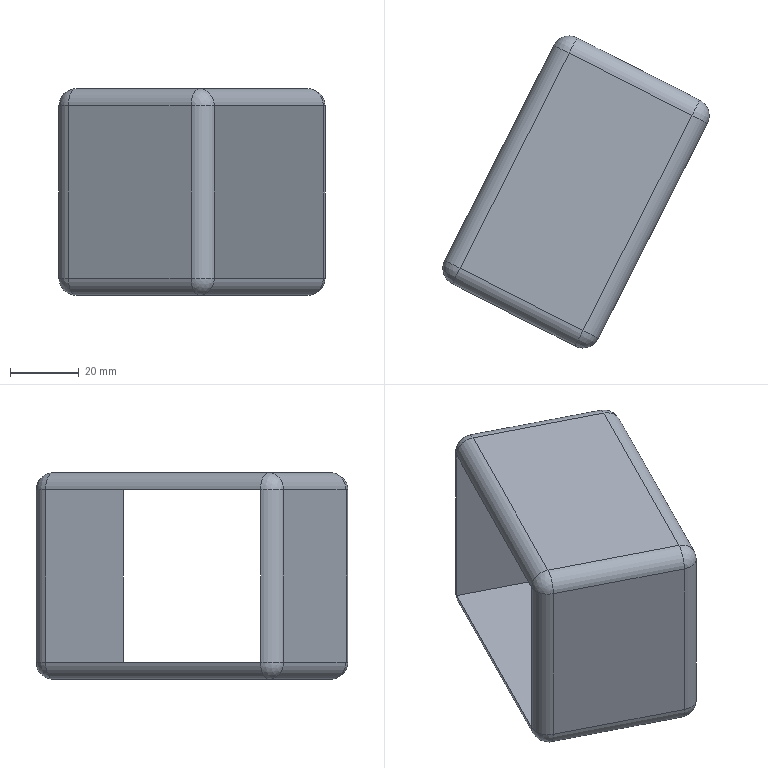Component | SolidWorks | FrameAssemblyDrawing11111-1_Part5ConnectingSleeve-1 | 1 solid | 28 faces | box 77.33 x 90.52 x 60 mm | volume 61090 mm3 | cylinder 12 | sphere 8 | plane 8 | commonest cylinder face diameters 10 x12
STEP:
#1=COLOUR_RGB('',0.7922,0.8196,0.9333);
#2=FILL_AREA_STYLE_COLOUR('',#1);
#3=FILL_AREA_STYLE('',(#2));
#4=SURFACE_STYLE_FILL_AREA(#3);
#5=SURFACE_SIDE_STYLE('',(#4));
#6=SURFACE_STYLE_USAGE(.BOTH.,#5);
#7=PRESENTATION_STYLE_ASSIGNMENT((#6));
#8=CARTESIAN_POINT('',(-32.016,-14.083,42.755));
#9=VERTEX_POINT('',#8);
#10=CARTESIAN_POINT('',(-32.28,-14.169,42.755));
#11=VERTEX_POINT('',#10);
#12=CARTESIAN_POINT('',(-32.105,-14.258,42.755));
#13=DIRECTION('',(-0.,-0.,1.));
#14=DIRECTION('',(0.892,-0.4521,-0.));
#15=AXIS2_PLACEMENT_3D('',#12,#13,#14);
#16=CIRCLE('',#15,0.1969);
#17=EDGE_CURVE('',#9,#11,#16,.T.);
#18=ORIENTED_EDGE('',*,*,#17,.F.);
#19=CARTESIAN_POINT('',(-32.016,-14.083,40.786));
#20=VERTEX_POINT('',#19);
#21=CARTESIAN_POINT('',(-32.016,-14.083,42.952));
#22=DIRECTION('',(-0.,-0.,1.));
#23=VECTOR('',#22,39.37);
#24=LINE('',#21,#23);
#25=EDGE_CURVE('',#20,#9,#24,.T.);
#26=ORIENTED_EDGE('',*,*,#25,.F.);
#27=CARTESIAN_POINT('',(-32.28,-14.169,40.786));
#28=VERTEX_POINT('',#27);
#29=CARTESIAN_POINT('',(-32.105,-14.258,40.786));
#30=DIRECTION('',(-0.,-0.,1.));
#31=DIRECTION('',(0.892,-0.4521,-0.));
#32=AXIS2_PLACEMENT_3D('',#29,#30,#31);
#33=CIRCLE('',#32,0.1969);
#34=EDGE_CURVE('',#20,#28,#33,.T.);
#35=ORIENTED_EDGE('',*,*,#34,.T.);
#36=CARTESIAN_POINT('',(-32.28,-14.169,42.952));
#37=DIRECTION('',(0.,0.,-1.));
#38=VECTOR('',#37,39.37);
#39=LINE('',#36,#38);
#40=EDGE_CURVE('',#11,#28,#39,.T.);
#41=ORIENTED_EDGE('',*,*,#40,.F.);
#42=EDGE_LOOP('',(#18,#26,#35,#41));
#43=FACE_OUTER_BOUND('',#42,.T.);
#44=CARTESIAN_POINT('',(-32.105,-14.258,42.952));
#45=DIRECTION('',(0.,0.,-1.));
#46=DIRECTION('',(-0.892,0.4521,0.));
#47=AXIS2_PLACEMENT_3D('',#44,#45,#46);
#48=CYLINDRICAL_SURFACE('',#47,0.1969);
#49=ADVANCED_FACE('',(#43),#48,.T.);
#50=ORIENTED_EDGE('',*,*,#34,.F.);
#51=CARTESIAN_POINT('',(-32.105,-14.258,40.589));
#52=VERTEX_POINT('',#51);
#53=CARTESIAN_POINT('',(-32.105,-14.258,40.786));
#54=DIRECTION('',(0.892,-0.4521,-0.));
#55=DIRECTION('',(-0.,-0.,1.));
#56=AXIS2_PLACEMENT_3D('',#53,#54,#55);
#57=CIRCLE('',#56,0.1969);
#58=EDGE_CURVE('',#52,#20,#57,.T.);
#59=ORIENTED_EDGE('',*,*,#58,.F.);
#60=CARTESIAN_POINT('',(-32.105,-14.258,40.786));
#61=DIRECTION('',(0.4521,0.892,0.));
#62=DIRECTION('',(-0.,-0.,1.));
#63=AXIS2_PLACEMENT_3D('',#60,#61,#62);
#64=CIRCLE('',#63,0.1969);
#65=EDGE_CURVE('',#52,#28,#64,.T.);
#66=ORIENTED_EDGE('',*,*,#65,.T.);
#67=EDGE_LOOP('',(#50,#59,#66));
#68=FACE_OUTER_BOUND('',#67,.T.);
#69=CARTESIAN_POINT('',(-32.105,-14.258,40.786));
#70=DIRECTION('',(0.4521,0.892,0.));
#71=DIRECTION('',(-0.,-0.,1.));
#72=AXIS2_PLACEMENT_3D('',#69,#70,#71);
#73=SPHERICAL_SURFACE('',#72,0.1969);
#74=ADVANCED_FACE('',(#68),#73,.T.);
#75=ORIENTED_EDGE('',*,*,#65,.F.);
#76=CARTESIAN_POINT('',(-33.351,-16.717,40.589));
#77=VERTEX_POINT('',#76);
#78=CARTESIAN_POINT('',(-32.016,-14.083,40.589));
#79=DIRECTION('',(0.4521,0.892,0.));
#80=VECTOR('',#79,39.37);
#81=LINE('',#78,#80);
#82=EDGE_CURVE('',#77,#52,#81,.T.);
#83=ORIENTED_EDGE('',*,*,#82,.F.);
#84=CARTESIAN_POINT('',(-33.526,-16.628,40.786));
#85=VERTEX_POINT('',#84);
#86=CARTESIAN_POINT('',(-33.351,-16.717,40.786));
#87=DIRECTION('',(0.4521,0.892,0.));
#88=DIRECTION('',(-0.,-0.,1.));
#89=AXIS2_PLACEMENT_3D('',#86,#87,#88);
#90=CIRCLE('',#89,0.1969);
#91=EDGE_CURVE('',#77,#85,#90,.T.);
#92=ORIENTED_EDGE('',*,*,#91,.T.);
#93=CARTESIAN_POINT('',(-32.191,-13.994,40.786));
#94=DIRECTION('',(-0.4521,-0.892,-0.));
#95=VECTOR('',#94,39.37);
#96=LINE('',#93,#95);
#97=EDGE_CURVE('',#28,#85,#96,.T.);
#98=ORIENTED_EDGE('',*,*,#97,.F.);
#99=EDGE_LOOP('',(#75,#83,#92,#98));
#100=FACE_OUTER_BOUND('',#99,.T.);
#101=CARTESIAN_POINT('',(-32.016,-14.083,40.786));
#102=DIRECTION('',(-0.4521,-0.892,-0.));
#103=DIRECTION('',(0.,0.,-1.));
#104=AXIS2_PLACEMENT_3D('',#101,#102,#103);
#105=CYLINDRICAL_SURFACE('',#104,0.1969);
#106=ADVANCED_FACE('',(#100),#105,.T.);
#107=ORIENTED_EDGE('',*,*,#91,.F.);
#108=CARTESIAN_POINT('',(-33.44,-16.892,40.786));
#109=VERTEX_POINT('',#108);
#110=CARTESIAN_POINT('',(-33.351,-16.717,40.786));
#111=DIRECTION('',(0.892,-0.4521,-0.));
#112=DIRECTION('',(-0.,-0.,1.));
#113=AXIS2_PLACEMENT_3D('',#110,#111,#112);
#114=CIRCLE('',#113,0.1969);
#115=EDGE_CURVE('',#109,#77,#114,.T.);
#116=ORIENTED_EDGE('',*,*,#115,.F.);
#117=CARTESIAN_POINT('',(-33.351,-16.717,40.786));
#118=DIRECTION('',(0.,0.,-1.));
#119=DIRECTION('',(-0.892,0.4521,0.));
#120=AXIS2_PLACEMENT_3D('',#117,#118,#119);
#121=CIRCLE('',#120,0.1969);
#122=EDGE_CURVE('',#109,#85,#121,.T.);
#123=ORIENTED_EDGE('',*,*,#122,.T.);
#124=EDGE_LOOP('',(#107,#116,#123));
#125=FACE_OUTER_BOUND('',#124,.T.);
#126=CARTESIAN_POINT('',(-33.351,-16.717,40.786));
#127=DIRECTION('',(0.4521,0.892,0.));
#128=DIRECTION('',(-0.,-0.,1.));
#129=AXIS2_PLACEMENT_3D('',#126,#127,#128);
#130=SPHERICAL_SURFACE('',#129,0.1969);
#131=ADVANCED_FACE('',(#125),#130,.T.);
#132=ORIENTED_EDGE('',*,*,#122,.F.);
#133=CARTESIAN_POINT('',(-33.44,-16.892,42.755));
#134=VERTEX_POINT('',#133);
#135=CARTESIAN_POINT('',(-33.44,-16.892,40.589));
#136=DIRECTION('',(0.,0.,-1.));
#137=VECTOR('',#136,39.37);
#138=LINE('',#135,#137);
#139=EDGE_CURVE('',#134,#109,#138,.T.);
#140=ORIENTED_EDGE('',*,*,#139,.F.);
#141=CARTESIAN_POINT('',(-33.526,-16.628,42.755));
#142=VERTEX_POINT('',#141);
#143=CARTESIAN_POINT('',(-33.351,-16.717,42.755));
#144=DIRECTION('',(0.,0.,-1.));
#145=DIRECTION('',(-0.892,0.4521,0.));
#146=AXIS2_PLACEMENT_3D('',#143,#144,#145);
#147=CIRCLE('',#146,0.1969);
#148=EDGE_CURVE('',#134,#142,#147,.T.);
#149=ORIENTED_EDGE('',*,*,#148,.T.);
#150=CARTESIAN_POINT('',(-33.526,-16.628,40.589));
#151=DIRECTION('',(-0.,-0.,1.));
#152=VECTOR('',#151,39.37);
#153=LINE('',#150,#152);
#154=EDGE_CURVE('',#85,#142,#153,.T.);
#155=ORIENTED_EDGE('',*,*,#154,.F.);
#156=EDGE_LOOP('',(#132,#140,#149,#155));
#157=FACE_OUTER_BOUND('',#156,.T.);
#158=CARTESIAN_POINT('',(-33.351,-16.717,40.589));
#159=DIRECTION('',(-0.,-0.,1.));
#160=DIRECTION('',(-0.4521,-0.892,-0.));
#161=AXIS2_PLACEMENT_3D('',#158,#159,#160);
#162=CYLINDRICAL_SURFACE('',#161,0.1969);
#163=ADVANCED_FACE('',(#157),#162,.T.);
#164=ORIENTED_EDGE('',*,*,#148,.F.);
#165=CARTESIAN_POINT('',(-33.351,-16.717,42.952));
#166=VERTEX_POINT('',#165);
#167=CARTESIAN_POINT('',(-33.351,-16.717,42.755));
#168=DIRECTION('',(0.892,-0.4521,-0.));
#169=DIRECTION('',(-0.,-0.,1.));
#170=AXIS2_PLACEMENT_3D('',#167,#168,#169);
#171=CIRCLE('',#170,0.1969);
#172=EDGE_CURVE('',#166,#134,#171,.T.);
#173=ORIENTED_EDGE('',*,*,#172,.F.);
#174=CARTESIAN_POINT('',(-33.351,-16.717,42.755));
#175=DIRECTION('',(-0.4521,-0.892,-0.));
#176=DIRECTION('',(0.,0.,-1.));
#177=AXIS2_PLACEMENT_3D('',#174,#175,#176);
#178=CIRCLE('',#177,0.1969);
#179=EDGE_CURVE('',#166,#142,#178,.T.);
#180=ORIENTED_EDGE('',*,*,#179,.T.);
#181=EDGE_LOOP('',(#164,#173,#180));
#182=FACE_OUTER_BOUND('',#181,.T.);
#183=CARTESIAN_POINT('',(-33.351,-16.717,42.755));
#184=DIRECTION('',(0.4521,0.892,0.));
#185=DIRECTION('',(-0.,-0.,1.));
#186=AXIS2_PLACEMENT_3D('',#183,#184,#185);
#187=SPHERICAL_SURFACE('',#186,0.1969);
#188=ADVANCED_FACE('',(#182),#187,.T.);
#189=ORIENTED_EDGE('',*,*,#179,.F.);
#190=CARTESIAN_POINT('',(-32.105,-14.258,42.952));
#191=VERTEX_POINT('',#190);
#192=CARTESIAN_POINT('',(-33.44,-16.892,42.952));
#193=DIRECTION('',(-0.4521,-0.892,-0.));
#194=VECTOR('',#193,39.37);
#195=LINE('',#192,#194);
#196=EDGE_CURVE('',#191,#166,#195,.T.);
#197=ORIENTED_EDGE('',*,*,#196,.F.);
#198=CARTESIAN_POINT('',(-32.105,-14.258,42.755));
#199=DIRECTION('',(-0.4521,-0.892,-0.));
#200=DIRECTION('',(0.,0.,-1.));
#201=AXIS2_PLACEMENT_3D('',#198,#199,#200);
#202=CIRCLE('',#201,0.1969);
#203=EDGE_CURVE('',#191,#11,#202,.T.);
#204=ORIENTED_EDGE('',*,*,#203,.T.);
#205=CARTESIAN_POINT('',(-33.615,-16.803,42.755));
#206=DIRECTION('',(0.4521,0.892,0.));
#207=VECTOR('',#206,39.37);
#208=LINE('',#205,#207);
#209=EDGE_CURVE('',#142,#11,#208,.T.);
#210=ORIENTED_EDGE('',*,*,#209,.F.);
#211=EDGE_LOOP('',(#189,#197,#204,#210));
#212=FACE_OUTER_BOUND('',#211,.T.);
#213=CARTESIAN_POINT('',(-33.44,-16.892,42.755));
#214=DIRECTION('',(0.4521,0.892,0.));
#215=DIRECTION('',(-0.,-0.,1.));
#216=AXIS2_PLACEMENT_3D('',#213,#214,#215);
#217=CYLINDRICAL_SURFACE('',#216,0.1969);
#218=ADVANCED_FACE('',(#212),#217,.T.);
#219=CARTESIAN_POINT('',(-32.105,-14.258,42.755));
#220=DIRECTION('',(0.892,-0.4521,-0.));
#221=DIRECTION('',(-0.,-0.,1.));
#222=AXIS2_PLACEMENT_3D('',#219,#220,#221);
#223=CIRCLE('',#222,0.1969);
#224=EDGE_CURVE('',#9,#191,#223,.T.);
#225=ORIENTED_EDGE('',*,*,#224,.F.);
#226=ORIENTED_EDGE('',*,*,#17,.T.);
#227=ORIENTED_EDGE('',*,*,#203,.F.);
#228=EDGE_LOOP('',(#225,#226,#227));
#229=FACE_OUTER_BOUND('',#228,.T.);
#230=CARTESIAN_POINT('',(-32.105,-14.258,42.755));
#231=DIRECTION('',(0.4521,0.892,0.));
#232=DIRECTION('',(-0.,-0.,1.));
#233=AXIS2_PLACEMENT_3D('',#230,#231,#232);
#234=SPHERICAL_SURFACE('',#233,0.1969);
#235=ADVANCED_FACE('',(#229),#234,.T.);
#236=CARTESIAN_POINT('',(-30.611,-14.795,40.786));
#237=VERTEX_POINT('',#236);
#238=CARTESIAN_POINT('',(-30.525,-15.059,40.786));
#239=VERTEX_POINT('',#238);
#240=CARTESIAN_POINT('',(-30.7,-14.97,40.786));
#241=DIRECTION('',(0.,0.,-1.));
#242=DIRECTION('',(-0.892,0.4521,0.));
#243=AXIS2_PLACEMENT_3D('',#240,#241,#242);
#244=CIRCLE('',#243,0.1969);
#245=EDGE_CURVE('',#237,#239,#244,.T.);
#246=ORIENTED_EDGE('',*,*,#245,.F.);
#247=CARTESIAN_POINT('',(-30.611,-14.795,42.755));
#248=VERTEX_POINT('',#247);
#249=CARTESIAN_POINT('',(-30.611,-14.795,42.952));
#250=DIRECTION('',(0.,0.,-1.));
#251=VECTOR('',#250,39.37);
#252=LINE('',#249,#251);
#253=EDGE_CURVE('',#248,#237,#252,.T.);
#254=ORIENTED_EDGE('',*,*,#253,.F.);
#255=CARTESIAN_POINT('',(-30.525,-15.059,42.755));
#256=VERTEX_POINT('',#255);
#257=CARTESIAN_POINT('',(-30.7,-14.97,42.755));
#258=DIRECTION('',(0.,0.,-1.));
#259=DIRECTION('',(-0.892,0.4521,0.));
#260=AXIS2_PLACEMENT_3D('',#257,#258,#259);
#261=CIRCLE('',#260,0.1969);
#262=EDGE_CURVE('',#248,#256,#261,.T.);
#263=ORIENTED_EDGE('',*,*,#262,.T.);
#264=CARTESIAN_POINT('',(-30.525,-15.059,40.376));
#265=DIRECTION('',(-0.,-0.,1.));
#266=VECTOR('',#265,39.37);
#267=LINE('',#264,#266);
#268=EDGE_CURVE('',#239,#256,#267,.T.);
#269=ORIENTED_EDGE('',*,*,#268,.F.);
#270=EDGE_LOOP('',(#246,#254,#263,#269));
#271=FACE_OUTER_BOUND('',#270,.T.);
#272=CARTESIAN_POINT('',(-30.7,-14.97,42.952));
#273=DIRECTION('',(0.,0.,-1.));
#274=DIRECTION('',(-0.892,0.4521,0.));
#275=AXIS2_PLACEMENT_3D('',#272,#273,#274);
#276=CYLINDRICAL_SURFACE('',#275,0.1969);
#277=ADVANCED_FACE('',(#271),#276,.T.);
#278=ORIENTED_EDGE('',*,*,#262,.F.);
#279=CARTESIAN_POINT('',(-30.7,-14.97,42.952));
#280=VERTEX_POINT('',#279);
#281=CARTESIAN_POINT('',(-30.7,-14.97,42.755));
#282=DIRECTION('',(-0.892,0.4521,0.));
#283=DIRECTION('',(-0.,-0.,1.));
#284=AXIS2_PLACEMENT_3D('',#281,#282,#283);
#285=CIRCLE('',#284,0.1969);
#286=EDGE_CURVE('',#280,#248,#285,.T.);
#287=ORIENTED_EDGE('',*,*,#286,.F.);
#288=CARTESIAN_POINT('',(-30.7,-14.97,42.755));
#289=DIRECTION('',(0.4521,0.892,0.));
#290=DIRECTION('',(-0.,-0.,1.));
#291=AXIS2_PLACEMENT_3D('',#288,#289,#290);
#292=CIRCLE('',#291,0.1969);
#293=EDGE_CURVE('',#280,#256,#292,.T.);
#294=ORIENTED_EDGE('',*,*,#293,.T.);
#295=EDGE_LOOP('',(#278,#287,#294));
#296=FACE_OUTER_BOUND('',#295,.T.);
#297=CARTESIAN_POINT('',(-30.7,-14.97,42.755));
#298=DIRECTION('',(0.4521,0.892,0.));
#299=DIRECTION('',(-0.,-0.,1.));
#300=AXIS2_PLACEMENT_3D('',#297,#298,#299);
#301=SPHERICAL_SURFACE('',#300,0.1969);
#302=ADVANCED_FACE('',(#296),#301,.T.);
#303=ORIENTED_EDGE('',*,*,#293,.F.);
#304=CARTESIAN_POINT('',(-31.946,-17.429,42.952));
#305=VERTEX_POINT('',#304);
#306=CARTESIAN_POINT('',(-32.035,-17.604,42.952));
#307=DIRECTION('',(0.4521,0.892,0.));
#308=VECTOR('',#307,39.37);
#309=LINE('',#306,#308);
#310=EDGE_CURVE('',#305,#280,#309,.T.);
#311=ORIENTED_EDGE('',*,*,#310,.F.);
#312=CARTESIAN_POINT('',(-31.771,-17.518,42.755));
#313=VERTEX_POINT('',#312);
#314=CARTESIAN_POINT('',(-31.946,-17.429,42.755));
#315=DIRECTION('',(0.4521,0.892,0.));
#316=DIRECTION('',(-0.,-0.,1.));
#317=AXIS2_PLACEMENT_3D('',#314,#315,#316);
#318=CIRCLE('',#317,0.1969);
#319=EDGE_CURVE('',#305,#313,#318,.T.);
#320=ORIENTED_EDGE('',*,*,#319,.T.);
#321=CARTESIAN_POINT('',(-31.592,-17.165,42.755));
#322=DIRECTION('',(-0.4521,-0.892,-0.));
#323=VECTOR('',#322,39.37);
#324=LINE('',#321,#323);
#325=EDGE_CURVE('',#256,#313,#324,.T.);
#326=ORIENTED_EDGE('',*,*,#325,.F.);
#327=EDGE_LOOP('',(#303,#311,#320,#326));
#328=FACE_OUTER_BOUND('',#327,.T.);
#329=CARTESIAN_POINT('',(-32.035,-17.604,42.755));
#330=DIRECTION('',(0.4521,0.892,0.));
#331=DIRECTION('',(-0.,-0.,1.));
#332=AXIS2_PLACEMENT_3D('',#329,#330,#331);
#333=CYLINDRICAL_SURFACE('',#332,0.1969);
#334=ADVANCED_FACE('',(#328),#333,.T.);
#335=ORIENTED_EDGE('',*,*,#319,.F.);
#336=CARTESIAN_POINT('',(-32.035,-17.604,42.755));
#337=VERTEX_POINT('',#336);
#338=CARTESIAN_POINT('',(-31.946,-17.429,42.755));
#339=DIRECTION('',(-0.892,0.4521,0.));
#340=DIRECTION('',(-0.,-0.,1.));
#341=AXIS2_PLACEMENT_3D('',#338,#339,#340);
#342=CIRCLE('',#341,0.1969);
#343=EDGE_CURVE('',#337,#305,#342,.T.);
#344=ORIENTED_EDGE('',*,*,#343,.F.);
#345=CARTESIAN_POINT('',(-31.946,-17.429,42.755));
#346=DIRECTION('',(-0.,-0.,1.));
#347=DIRECTION('',(0.892,-0.4521,-0.));
#348=AXIS2_PLACEMENT_3D('',#345,#346,#347);
#349=CIRCLE('',#348,0.1969);
#350=EDGE_CURVE('',#337,#313,#349,.T.);
#351=ORIENTED_EDGE('',*,*,#350,.T.);
#352=EDGE_LOOP('',(#335,#344,#351));
#353=FACE_OUTER_BOUND('',#352,.T.);
#354=CARTESIAN_POINT('',(-31.946,-17.429,42.755));
#355=DIRECTION('',(0.4521,0.892,0.));
#356=DIRECTION('',(-0.,-0.,1.));
#357=AXIS2_PLACEMENT_3D('',#354,#355,#356);
#358=SPHERICAL_SURFACE('',#357,0.1969);
#359=ADVANCED_FACE('',(#353),#358,.T.);
#360=ORIENTED_EDGE('',*,*,#350,.F.);
#361=CARTESIAN_POINT('',(-32.035,-17.604,40.786));
#362=VERTEX_POINT('',#361);
#363=CARTESIAN_POINT('',(-32.035,-17.604,40.589));
#364=DIRECTION('',(-0.,-0.,1.));
#365=VECTOR('',#364,39.37);
#366=LINE('',#363,#365);
#367=EDGE_CURVE('',#362,#337,#366,.T.);
#368=ORIENTED_EDGE('',*,*,#367,.F.);
#369=CARTESIAN_POINT('',(-31.771,-17.518,40.786));
#370=VERTEX_POINT('',#369);
#371=CARTESIAN_POINT('',(-31.946,-17.429,40.786));
#372=DIRECTION('',(-0.,-0.,1.));
#373=DIRECTION('',(0.892,-0.4521,-0.));
#374=AXIS2_PLACEMENT_3D('',#371,#372,#373);
#375=CIRCLE('',#374,0.1969);
#376=EDGE_CURVE('',#362,#370,#375,.T.);
#377=ORIENTED_EDGE('',*,*,#376,.T.);
#378=CARTESIAN_POINT('',(-31.771,-17.518,40.376));
#379=DIRECTION('',(0.,0.,-1.));
#380=VECTOR('',#379,39.37);
#381=LINE('',#378,#380);
#382=EDGE_CURVE('',#313,#370,#381,.T.);
#383=ORIENTED_EDGE('',*,*,#382,.F.);
#384=EDGE_LOOP('',(#360,#368,#377,#383));
#385=FACE_OUTER_BOUND('',#384,.T.);
#386=CARTESIAN_POINT('',(-31.946,-17.429,40.589));
#387=DIRECTION('',(-0.,-0.,1.));
#388=DIRECTION('',(-0.4521,-0.892,-0.));
#389=AXIS2_PLACEMENT_3D('',#386,#387,#388);
#390=CYLINDRICAL_SURFACE('',#389,0.1969);
#391=ADVANCED_FACE('',(#385),#390,.T.);
#392=ORIENTED_EDGE('',*,*,#376,.F.);
#393=CARTESIAN_POINT('',(-31.946,-17.429,40.589));
#394=VERTEX_POINT('',#393);
#395=CARTESIAN_POINT('',(-31.946,-17.429,40.786));
#396=DIRECTION('',(-0.892,0.4521,0.));
#397=DIRECTION('',(-0.,-0.,1.));
#398=AXIS2_PLACEMENT_3D('',#395,#396,#397);
#399=CIRCLE('',#398,0.1969);
#400=EDGE_CURVE('',#394,#362,#399,.T.);
#401=ORIENTED_EDGE('',*,*,#400,.F.);
#402=CARTESIAN_POINT('',(-31.946,-17.429,40.786));
#403=DIRECTION('',(-0.4521,-0.892,-0.));
#404=DIRECTION('',(0.,0.,-1.));
#405=AXIS2_PLACEMENT_3D('',#402,#403,#404);
#406=CIRCLE('',#405,0.1969);
#407=EDGE_CURVE('',#394,#370,#406,.T.);
#408=ORIENTED_EDGE('',*,*,#407,.T.);
#409=EDGE_LOOP('',(#392,#401,#408));
#410=FACE_OUTER_BOUND('',#409,.T.);
#411=CARTESIAN_POINT('',(-31.946,-17.429,40.786));
#412=DIRECTION('',(0.4521,0.892,0.));
#413=DIRECTION('',(-0.,-0.,1.));
#414=AXIS2_PLACEMENT_3D('',#411,#412,#413);
#415=SPHERICAL_SURFACE('',#414,0.1969);
#416=ADVANCED_FACE('',(#410),#415,.T.);
#417=ORIENTED_EDGE('',*,*,#407,.F.);
#418=CARTESIAN_POINT('',(-30.7,-14.97,40.589));
#419=VERTEX_POINT('',#418);
#420=CARTESIAN_POINT('',(-30.611,-14.795,40.589));
#421=DIRECTION('',(-0.4521,-0.892,-0.));
#422=VECTOR('',#421,39.37);
#423=LINE('',#420,#422);
#424=EDGE_CURVE('',#419,#394,#423,.T.);
#425=ORIENTED_EDGE('',*,*,#424,.F.);
#426=CARTESIAN_POINT('',(-30.7,-14.97,40.786));
#427=DIRECTION('',(-0.4521,-0.892,-0.));
#428=DIRECTION('',(0.,0.,-1.));
#429=AXIS2_PLACEMENT_3D('',#426,#427,#428);
#430=CIRCLE('',#429,0.1969);
#431=EDGE_CURVE('',#419,#239,#430,.T.);
#432=ORIENTED_EDGE('',*,*,#431,.T.);
#433=CARTESIAN_POINT('',(-31.592,-17.165,40.786));
#434=DIRECTION('',(0.4521,0.892,0.));
#435=VECTOR('',#434,39.37);
#436=LINE('',#433,#435);
#437=EDGE_CURVE('',#370,#239,#436,.T.);
#438=ORIENTED_EDGE('',*,*,#437,.F.);
#439=EDGE_LOOP('',(#417,#425,#432,#438));
#440=FACE_OUTER_BOUND('',#439,.T.);
#441=CARTESIAN_POINT('',(-30.611,-14.795,40.786));
#442=DIRECTION('',(-0.4521,-0.892,-0.));
#443=DIRECTION('',(0.,0.,-1.));
#444=AXIS2_PLACEMENT_3D('',#441,#442,#443);
#445=CYLINDRICAL_SURFACE('',#444,0.1969);
#446=ADVANCED_FACE('',(#440),#445,.T.);
#447=CARTESIAN_POINT('',(-30.7,-14.97,40.786));
#448=DIRECTION('',(-0.892,0.4521,0.));
#449=DIRECTION('',(-0.,-0.,1.));
#450=AXIS2_PLACEMENT_3D('',#447,#448,#449);
#451=CIRCLE('',#450,0.1969);
#452=EDGE_CURVE('',#237,#419,#451,.T.);
#453=ORIENTED_EDGE('',*,*,#452,.F.);
#454=ORIENTED_EDGE('',*,*,#245,.T.);
#455=ORIENTED_EDGE('',*,*,#431,.F.);
#456=EDGE_LOOP('',(#453,#454,#455));
#457=FACE_OUTER_BOUND('',#456,.T.);
#458=CARTESIAN_POINT('',(-30.7,-14.97,40.786));
#459=DIRECTION('',(0.4521,0.892,0.));
#460=DIRECTION('',(-0.,-0.,1.));
#461=AXIS2_PLACEMENT_3D('',#458,#459,#460);
#462=SPHERICAL_SURFACE('',#461,0.1969);
#463=ADVANCED_FACE('',(#457),#462,.T.);
#464=CARTESIAN_POINT('',(-30.525,-15.059,42.952));
#465=DIRECTION('',(-0.892,0.4521,0.));
#466=VECTOR('',#465,39.37);
#467=LINE('',#464,#466);
#468=EDGE_CURVE('',#280,#191,#467,.T.);
#469=ORIENTED_EDGE('',*,*,#468,.T.);
#470=ORIENTED_EDGE('',*,*,#196,.T.);
#471=CARTESIAN_POINT('',(-31.771,-17.518,42.952));
#472=DIRECTION('',(0.892,-0.4521,-0.));
#473=VECTOR('',#472,39.37);
#474=LINE('',#471,#473);
#475=EDGE_CURVE('',#166,#305,#474,.T.);
#476=ORIENTED_EDGE('',*,*,#475,.T.);
#477=ORIENTED_EDGE('',*,*,#310,.T.);
#478=EDGE_LOOP('',(#469,#470,#476,#477));
#479=FACE_OUTER_BOUND('',#478,.T.);
#480=CARTESIAN_POINT('',(-31.86,-17.693,42.952));
#481=DIRECTION('',(0.,0.,-1.));
#482=DIRECTION('',(-0.892,0.4521,0.));
#483=AXIS2_PLACEMENT_3D('',#480,#481,#482);
#484=PLANE('',#483);
#485=ADVANCED_FACE('',(#479),#484,.F.);
#486=CARTESIAN_POINT('',(-31.86,-17.693,42.755));
#487=DIRECTION('',(-0.892,0.4521,0.));
#488=VECTOR('',#487,39.37);
#489=LINE('',#486,#488);
#490=EDGE_CURVE('',#337,#134,#489,.T.);
#491=ORIENTED_EDGE('',*,*,#490,.T.);
#492=ORIENTED_EDGE('',*,*,#139,.T.);
#493=CARTESIAN_POINT('',(-31.86,-17.693,40.786));
#494=DIRECTION('',(0.892,-0.4521,-0.));
#495=VECTOR('',#494,39.37);
#496=LINE('',#493,#495);
#497=EDGE_CURVE('',#109,#362,#496,.T.);
#498=ORIENTED_EDGE('',*,*,#497,.T.);
#499=ORIENTED_EDGE('',*,*,#367,.T.);
#500=EDGE_LOOP('',(#491,#492,#498,#499));
#501=FACE_OUTER_BOUND('',#500,.T.);
#502=CARTESIAN_POINT('',(-31.86,-17.693,40.589));
#503=DIRECTION('',(0.4521,0.892,0.));
#504=DIRECTION('',(-0.,-0.,1.));
#505=AXIS2_PLACEMENT_3D('',#502,#503,#504);
#506=PLANE('',#505);
#507=ADVANCED_FACE('',(#501),#506,.F.);
#508=CARTESIAN_POINT('',(-31.771,-17.518,40.589));
#509=DIRECTION('',(-0.892,0.4521,0.));
#510=VECTOR('',#509,39.37);
#511=LINE('',#508,#510);
#512=EDGE_CURVE('',#394,#77,#511,.T.);
#513=ORIENTED_EDGE('',*,*,#512,.T.);
#514=ORIENTED_EDGE('',*,*,#82,.T.);
#515=CARTESIAN_POINT('',(-30.525,-15.059,40.589));
#516=DIRECTION('',(0.892,-0.4521,-0.));
#517=VECTOR('',#516,39.37);
#518=LINE('',#515,#517);
#519=EDGE_CURVE('',#52,#419,#518,.T.);
#520=ORIENTED_EDGE('',*,*,#519,.T.);
#521=ORIENTED_EDGE('',*,*,#424,.T.);
#522=EDGE_LOOP('',(#513,#514,#520,#521));
#523=FACE_OUTER_BOUND('',#522,.T.);
#524=CARTESIAN_POINT('',(-30.436,-14.884,40.589));
#525=DIRECTION('',(-0.,-0.,1.));
#526=DIRECTION('',(-0.4521,-0.892,-0.));
#527=AXIS2_PLACEMENT_3D('',#524,#525,#526);
#528=PLANE('',#527);
#529=ADVANCED_FACE('',(#523),#528,.F.);
#530=CARTESIAN_POINT('',(-30.436,-14.884,40.786));
#531=DIRECTION('',(-0.892,0.4521,0.));
#532=VECTOR('',#531,39.37);
#533=LINE('',#530,#532);
#534=EDGE_CURVE('',#237,#20,#533,.T.);
#535=ORIENTED_EDGE('',*,*,#534,.T.);
#536=ORIENTED_EDGE('',*,*,#25,.T.);
#537=CARTESIAN_POINT('',(-30.436,-14.884,42.755));
#538=DIRECTION('',(0.892,-0.4521,-0.));
#539=VECTOR('',#538,39.37);
#540=LINE('',#537,#539);
#541=EDGE_CURVE('',#9,#248,#540,.T.);
#542=ORIENTED_EDGE('',*,*,#541,.T.);
#543=ORIENTED_EDGE('',*,*,#253,.T.);
#544=EDGE_LOOP('',(#535,#536,#542,#543));
#545=FACE_OUTER_BOUND('',#544,.T.);
#546=CARTESIAN_POINT('',(-30.436,-14.884,42.952));
#547=DIRECTION('',(-0.4521,-0.892,-0.));
#548=DIRECTION('',(0.,0.,-1.));
#549=AXIS2_PLACEMENT_3D('',#546,#547,#548);
#550=PLANE('',#549);
#551=ADVANCED_FACE('',(#545),#550,.F.);
#552=ORIENTED_EDGE('',*,*,#541,.F.);
#553=ORIENTED_EDGE('',*,*,#224,.T.);
#554=ORIENTED_EDGE('',*,*,#468,.F.);
#555=ORIENTED_EDGE('',*,*,#286,.T.);
#556=EDGE_LOOP('',(#552,#553,#554,#555));
#557=FACE_OUTER_BOUND('',#556,.T.);
#558=CARTESIAN_POINT('',(-30.525,-15.059,42.755));
#559=DIRECTION('',(-0.892,0.4521,0.));
#560=DIRECTION('',(-0.,-0.,1.));
#561=AXIS2_PLACEMENT_3D('',#558,#559,#560);
#562=CYLINDRICAL_SURFACE('',#561,0.1969);
#563=ADVANCED_FACE('',(#557),#562,.T.);
#564=ORIENTED_EDGE('',*,*,#497,.F.);
#565=ORIENTED_EDGE('',*,*,#115,.T.);
#566=ORIENTED_EDGE('',*,*,#512,.F.);
#567=ORIENTED_EDGE('',*,*,#400,.T.);
#568=EDGE_LOOP('',(#564,#565,#566,#567));
#569=FACE_OUTER_BOUND('',#568,.T.);
#570=CARTESIAN_POINT('',(-31.771,-17.518,40.786));
#571=DIRECTION('',(-0.892,0.4521,0.));
#572=DIRECTION('',(-0.,-0.,1.));
#573=AXIS2_PLACEMENT_3D('',#570,#571,#572);
#574=CYLINDRICAL_SURFACE('',#573,0.1969);
#575=ADVANCED_FACE('',(#569),#574,.T.);
#576=ORIENTED_EDGE('',*,*,#475,.F.);
#577=ORIENTED_EDGE('',*,*,#172,.T.);
#578=ORIENTED_EDGE('',*,*,#490,.F.);
#579=ORIENTED_EDGE('',*,*,#343,.T.);
#580=EDGE_LOOP('',(#576,#577,#578,#579));
#581=FACE_OUTER_BOUND('',#580,.T.);
#582=CARTESIAN_POINT('',(-31.771,-17.518,42.755));
#583=DIRECTION('',(-0.892,0.4521,0.));
#584=DIRECTION('',(-0.,-0.,1.));
#585=AXIS2_PLACEMENT_3D('',#582,#583,#584);
#586=CYLINDRICAL_SURFACE('',#585,0.1969);
#587=ADVANCED_FACE('',(#581),#586,.T.);
#588=ORIENTED_EDGE('',*,*,#519,.F.);
#589=ORIENTED_EDGE('',*,*,#58,.T.);
#590=ORIENTED_EDGE('',*,*,#534,.F.);
#591=ORIENTED_EDGE('',*,*,#452,.T.);
#592=EDGE_LOOP('',(#588,#589,#590,#591));
#593=FACE_OUTER_BOUND('',#592,.T.);
#594=CARTESIAN_POINT('',(-30.525,-15.059,40.786));
#595=DIRECTION('',(-0.892,0.4521,0.));
#596=DIRECTION('',(-0.,-0.,1.));
#597=AXIS2_PLACEMENT_3D('',#594,#595,#596);
#598=CYLINDRICAL_SURFACE('',#597,0.1969);
#599=ADVANCED_FACE('',(#593),#598,.T.);
#600=CARTESIAN_POINT('',(-30.525,-15.059,42.755));
#601=DIRECTION('',(-0.892,0.4521,0.));
#602=VECTOR('',#601,39.37);
#603=LINE('',#600,#602);
#604=EDGE_CURVE('',#256,#11,#603,.T.);
#605=ORIENTED_EDGE('',*,*,#604,.F.);
#606=ORIENTED_EDGE('',*,*,#325,.T.);
#607=CARTESIAN_POINT('',(-31.771,-17.518,42.755));
#608=DIRECTION('',(-0.892,0.4521,0.));
#609=VECTOR('',#608,39.37);
#610=LINE('',#607,#609);
#611=EDGE_CURVE('',#313,#142,#610,.T.);
#612=ORIENTED_EDGE('',*,*,#611,.T.);
#613=ORIENTED_EDGE('',*,*,#209,.T.);
#614=EDGE_LOOP('',(#605,#606,#612,#613));
#615=FACE_OUTER_BOUND('',#614,.T.);
#616=CARTESIAN_POINT('',(-31.86,-17.693,42.755));
#617=DIRECTION('',(0.,0.,-1.));
#618=DIRECTION('',(-0.892,0.4521,0.));
#619=AXIS2_PLACEMENT_3D('',#616,#617,#618);
#620=PLANE('',#619);
#621=ADVANCED_FACE('',(#615),#620,.T.);
#622=ORIENTED_EDGE('',*,*,#611,.F.);
#623=ORIENTED_EDGE('',*,*,#382,.T.);
#624=CARTESIAN_POINT('',(-31.771,-17.518,40.786));
#625=DIRECTION('',(-0.892,0.4521,0.));
#626=VECTOR('',#625,39.37);
#627=LINE('',#624,#626);
#628=EDGE_CURVE('',#370,#85,#627,.T.);
#629=ORIENTED_EDGE('',*,*,#628,.T.);
#630=ORIENTED_EDGE('',*,*,#154,.T.);
#631=EDGE_LOOP('',(#622,#623,#629,#630));
#632=FACE_OUTER_BOUND('',#631,.T.);
#633=CARTESIAN_POINT('',(-31.771,-17.518,40.589));
#634=DIRECTION('',(0.4521,0.892,0.));
#635=DIRECTION('',(-0.,-0.,1.));
#636=AXIS2_PLACEMENT_3D('',#633,#634,#635);
#637=PLANE('',#636);
#638=ADVANCED_FACE('',(#632),#637,.T.);
#639=ORIENTED_EDGE('',*,*,#628,.F.);
#640=ORIENTED_EDGE('',*,*,#437,.T.);
#641=CARTESIAN_POINT('',(-30.525,-15.059,40.786));
#642=DIRECTION('',(-0.892,0.4521,0.));
#643=VECTOR('',#642,39.37);
#644=LINE('',#641,#643);
#645=EDGE_CURVE('',#239,#28,#644,.T.);
#646=ORIENTED_EDGE('',*,*,#645,.T.);
#647=ORIENTED_EDGE('',*,*,#97,.T.);
#648=EDGE_LOOP('',(#639,#640,#646,#647));
#649=FACE_OUTER_BOUND('',#648,.T.);
#650=CARTESIAN_POINT('',(-30.436,-14.884,40.786));
#651=DIRECTION('',(-0.,-0.,1.));
#652=DIRECTION('',(-0.4521,-0.892,-0.));
#653=AXIS2_PLACEMENT_3D('',#650,#651,#652);
#654=PLANE('',#653);
#655=ADVANCED_FACE('',(#649),#654,.T.);
#656=ORIENTED_EDGE('',*,*,#645,.F.);
#657=ORIENTED_EDGE('',*,*,#268,.T.);
#658=ORIENTED_EDGE('',*,*,#604,.T.);
#659=ORIENTED_EDGE('',*,*,#40,.T.);
#660=EDGE_LOOP('',(#656,#657,#658,#659));
#661=FACE_OUTER_BOUND('',#660,.T.);
#662=CARTESIAN_POINT('',(-30.525,-15.059,42.952));
#663=DIRECTION('',(-0.4521,-0.892,-0.));
#664=DIRECTION('',(0.,0.,-1.));
#665=AXIS2_PLACEMENT_3D('',#662,#663,#664);
#666=PLANE('',#665);
#667=ADVANCED_FACE('',(#661),#666,.T.);
#668=CLOSED_SHELL('',(#49,#74,#106,#131,#163,#188,#218,#235,#277,#302,#334,#359,#391,#416,#446,#463,#485,#507,#529,#551,#563,#575,#587,#599,#621,#638,#655,#667));
#669=MANIFOLD_SOLID_BREP('',#668);
#670=STYLED_ITEM('',(#7),#669);
#671=(LENGTH_UNIT()NAMED_UNIT(*)SI_UNIT($,.METRE.));
#672=LENGTH_MEASURE_WITH_UNIT(LENGTH_MEASURE(0.0254),#671);
#673=DIMENSIONAL_EXPONENTS(1.,0.,0.,0.,0.,0.,0.);
#674=(CONVERSION_BASED_UNIT('',#672)LENGTH_UNIT()NAMED_UNIT(#673));
#675=UNCERTAINTY_MEASURE_WITH_UNIT(LENGTH_MEASURE(0.00001),#674,'','');
#676=(NAMED_UNIT(*)PLANE_ANGLE_UNIT()SI_UNIT($,.RADIAN.));
#677=(NAMED_UNIT(*)SI_UNIT($,.STERADIAN.)SOLID_ANGLE_UNIT());
#678=(GEOMETRIC_REPRESENTATION_CONTEXT(3)GLOBAL_UNCERTAINTY_ASSIGNED_CONTEXT((#675))GLOBAL_UNIT_ASSIGNED_CONTEXT((#674,#676,#677))REPRESENTATION_CONTEXT('',''));
#679=MECHANICAL_DESIGN_GEOMETRIC_PRESENTATION_REPRESENTATION('',(#670),#678);
#680=CARTESIAN_POINT('',(0.,0.,0.));
#681=DIRECTION('',(0.,0.,1.));
#682=DIRECTION('',(1.,0.,0.));
#683=AXIS2_PLACEMENT_3D('',#680,#681,#682);
#684=(LENGTH_UNIT()NAMED_UNIT(*)SI_UNIT($,.METRE.));
#685=LENGTH_MEASURE_WITH_UNIT(LENGTH_MEASURE(0.0254),#684);
#686=DIMENSIONAL_EXPONENTS(1.,0.,0.,0.,0.,0.,0.);
#687=(CONVERSION_BASED_UNIT('',#685)LENGTH_UNIT()NAMED_UNIT(#686));
#688=UNCERTAINTY_MEASURE_WITH_UNIT(LENGTH_MEASURE(0.00001),#687,'','');
#689=(NAMED_UNIT(*)PLANE_ANGLE_UNIT()SI_UNIT($,.RADIAN.));
#690=(NAMED_UNIT(*)SI_UNIT($,.STERADIAN.)SOLID_ANGLE_UNIT());
#691=(GEOMETRIC_REPRESENTATION_CONTEXT(3)GLOBAL_UNCERTAINTY_ASSIGNED_CONTEXT((#688))GLOBAL_UNIT_ASSIGNED_CONTEXT((#687,#689,#690))REPRESENTATION_CONTEXT('',''));
#692=ADVANCED_BREP_SHAPE_REPRESENTATION('',(#669,#683),#691);
#693=PRESENTATION_LAYER_ASSIGNMENT('','',(#670));